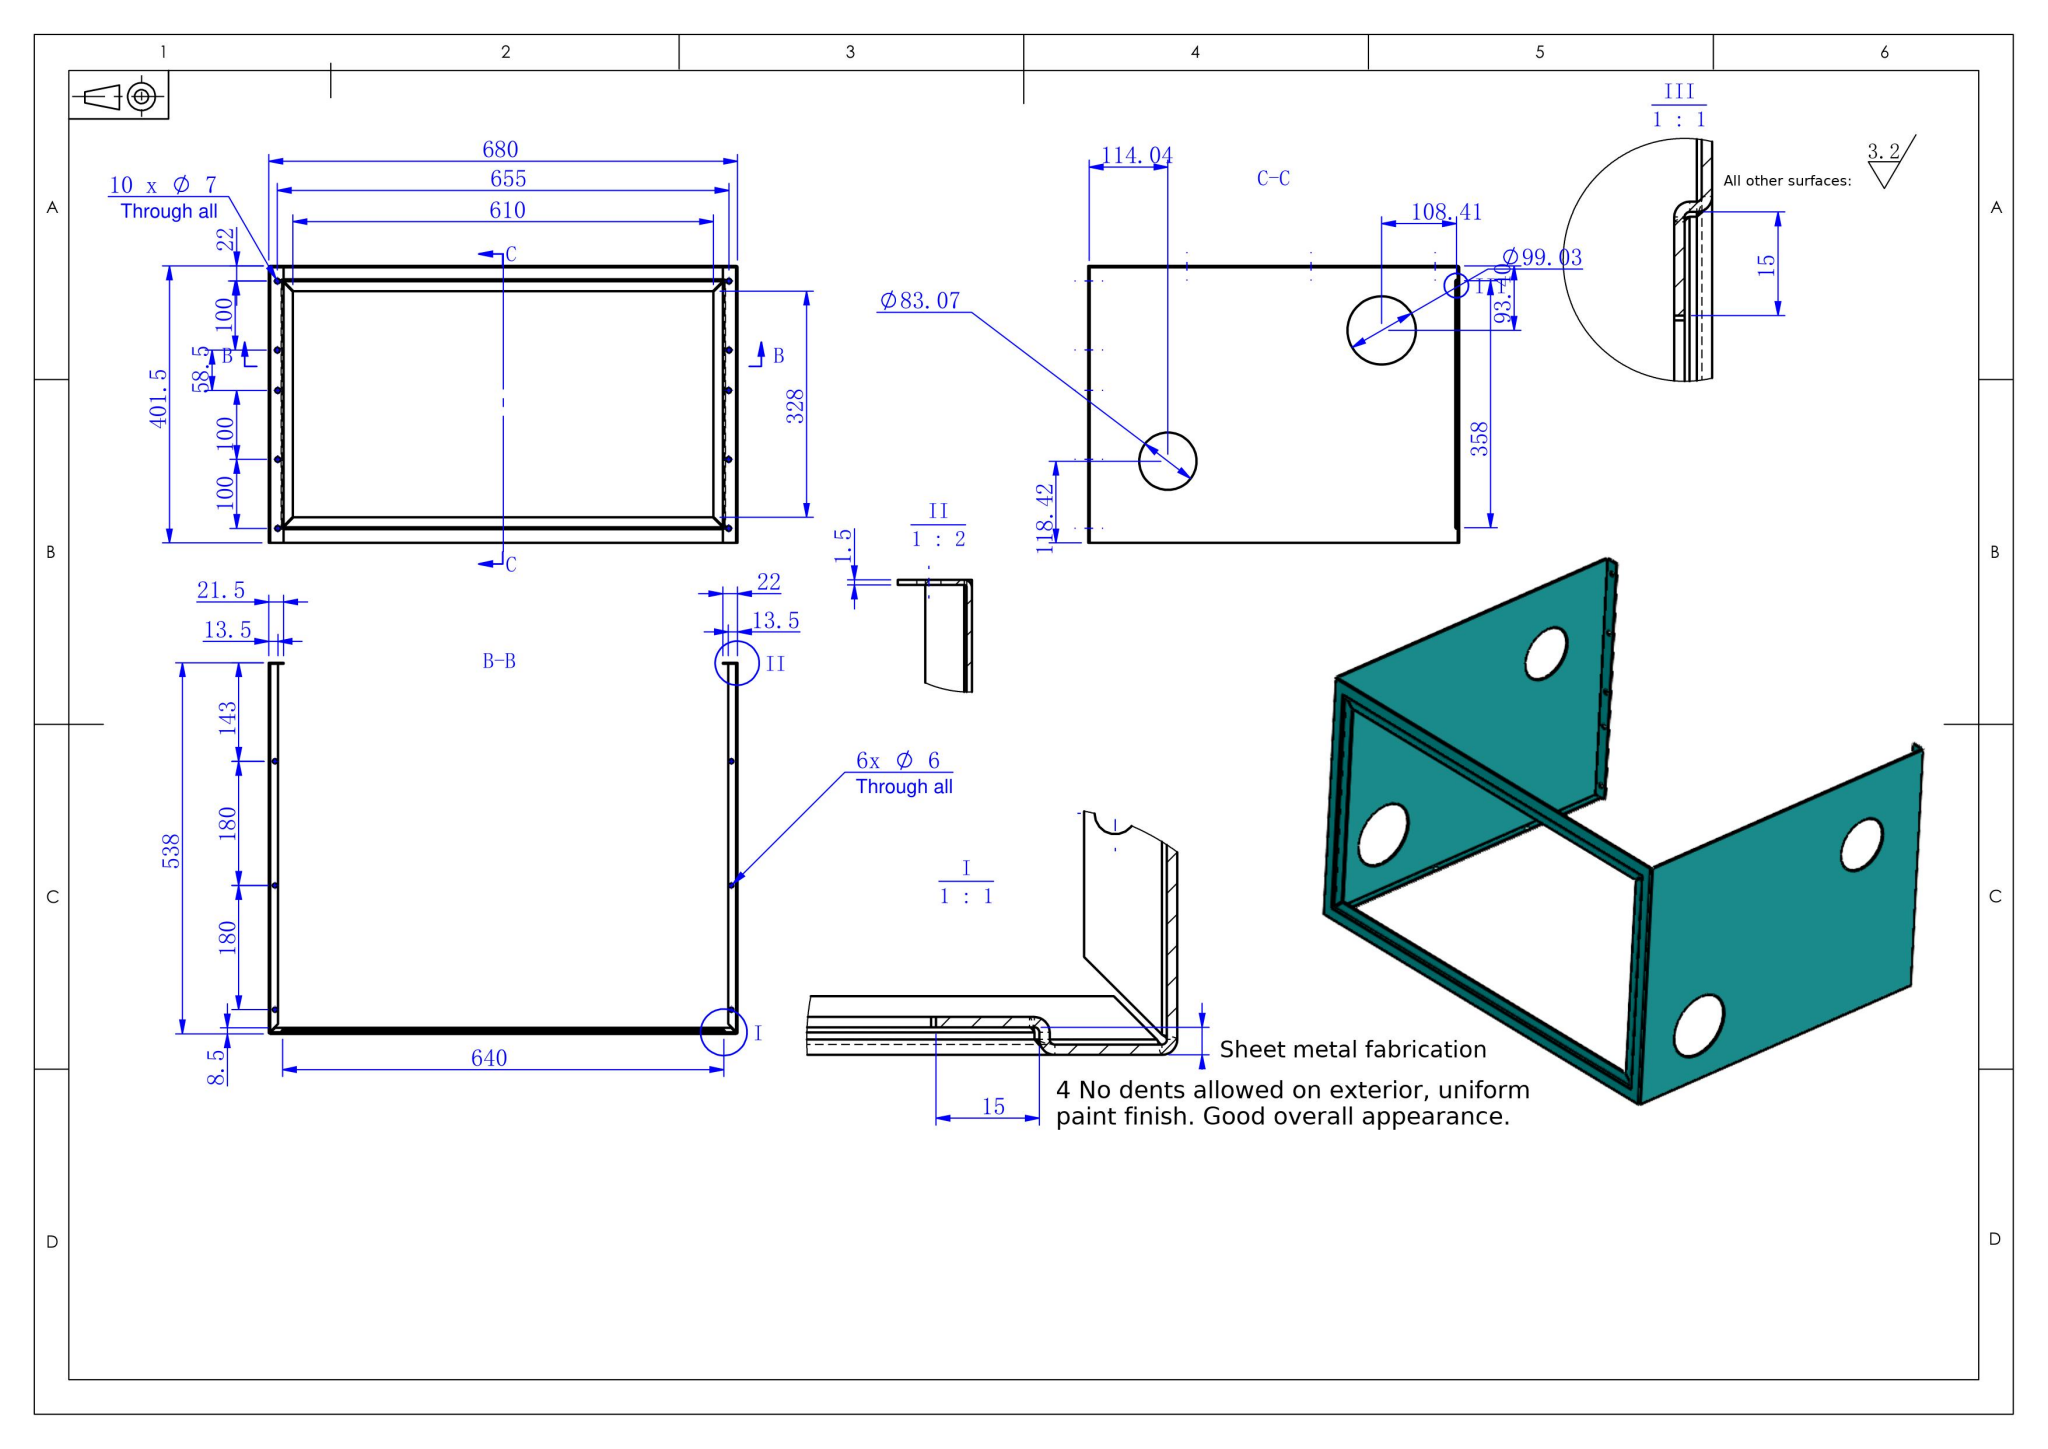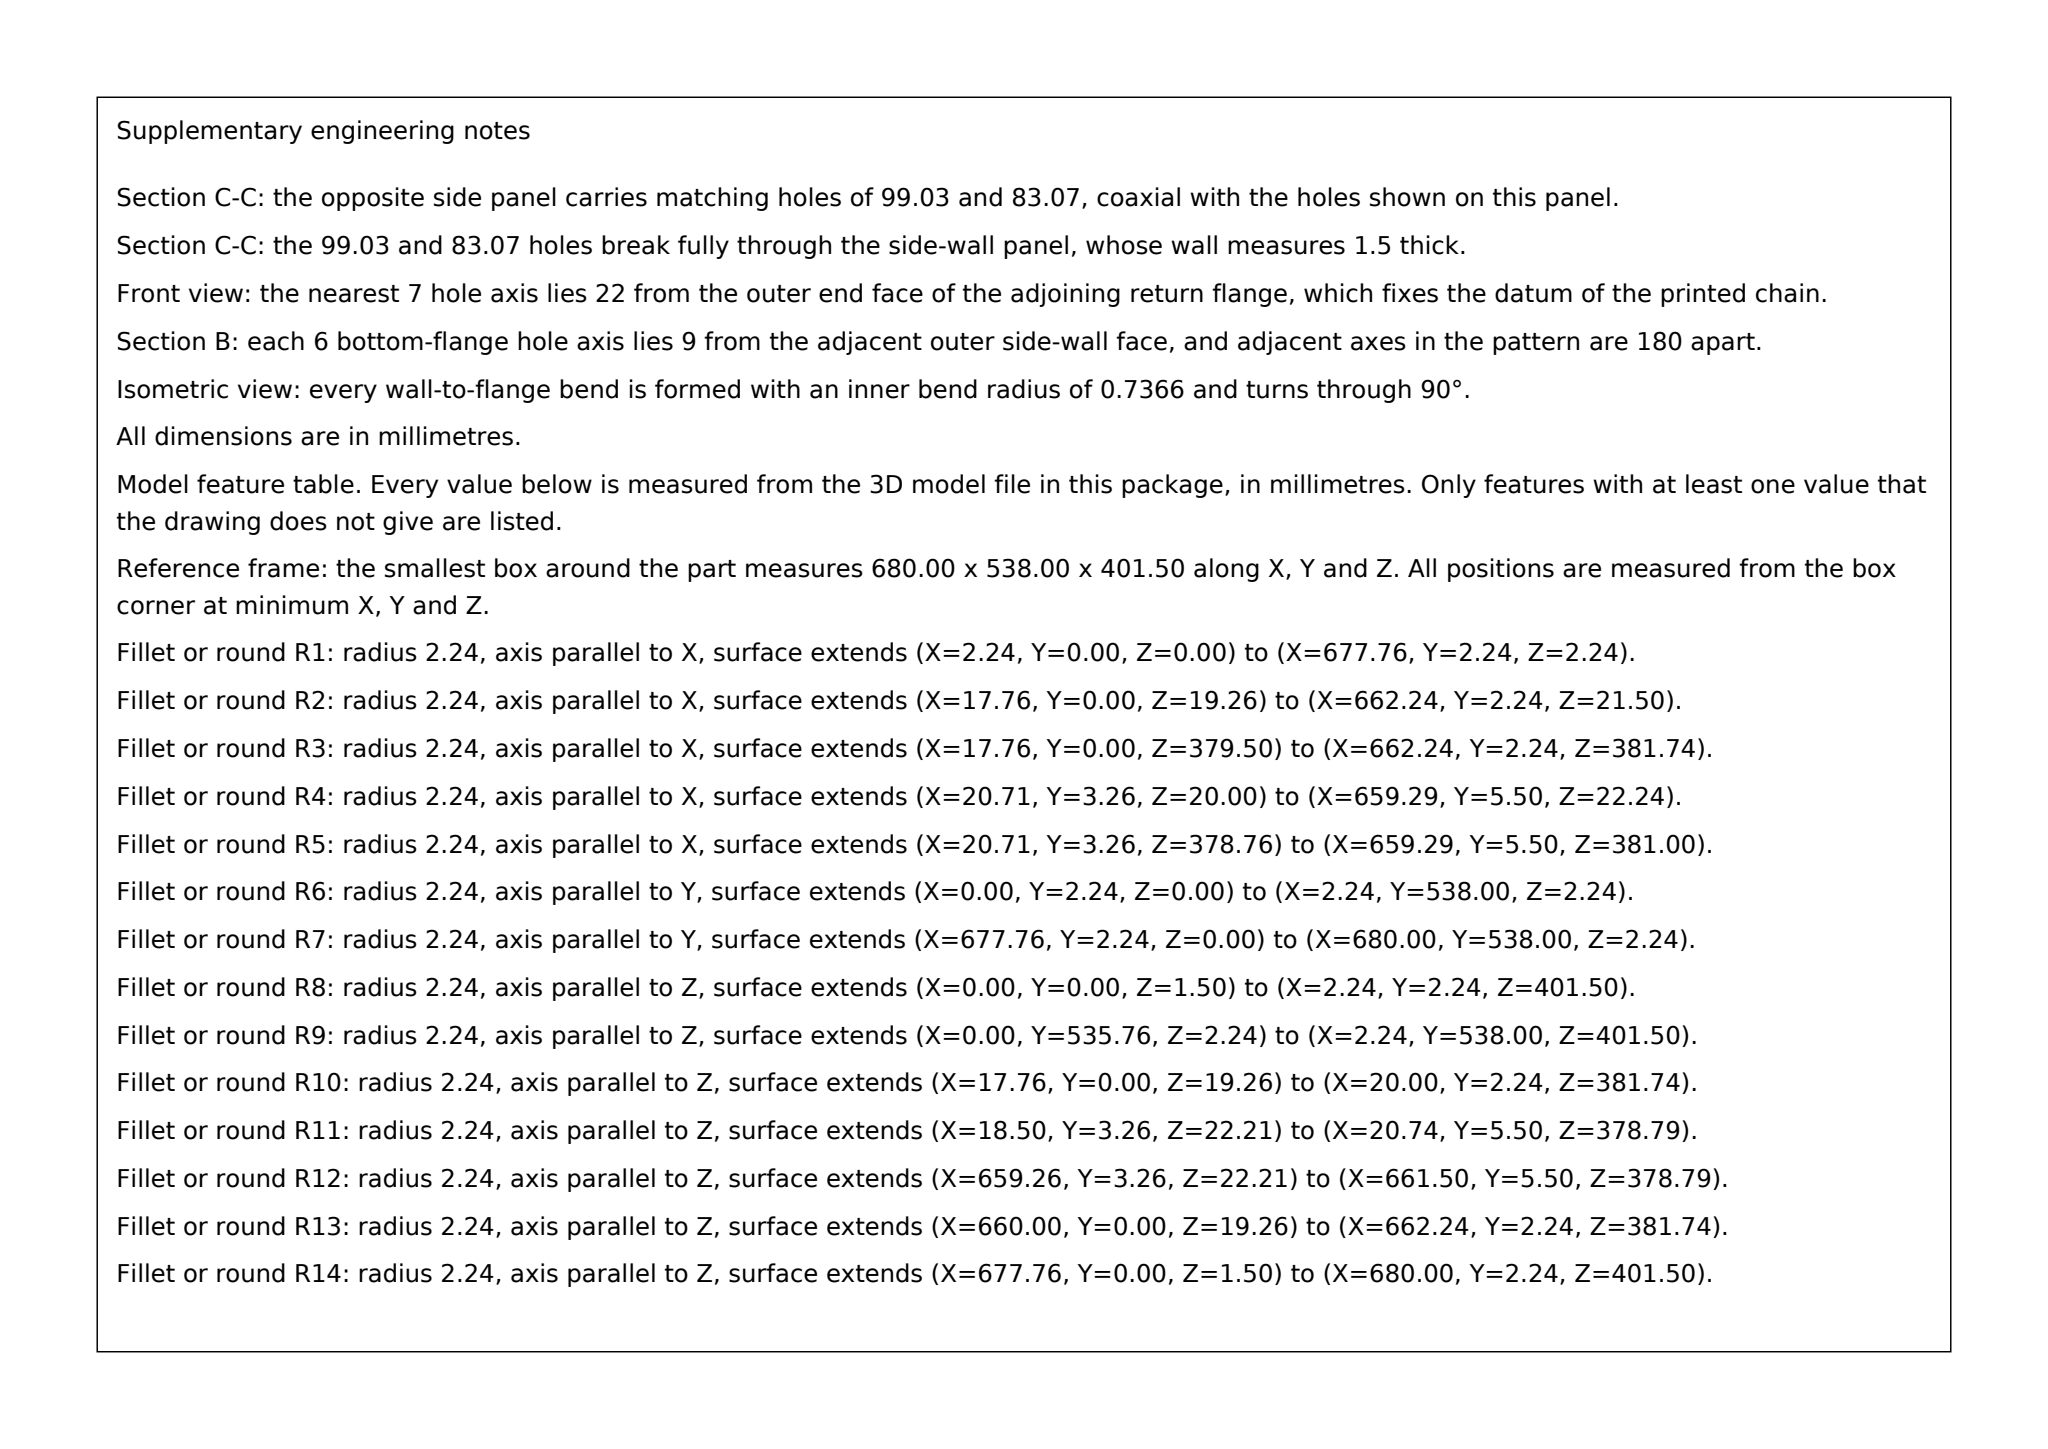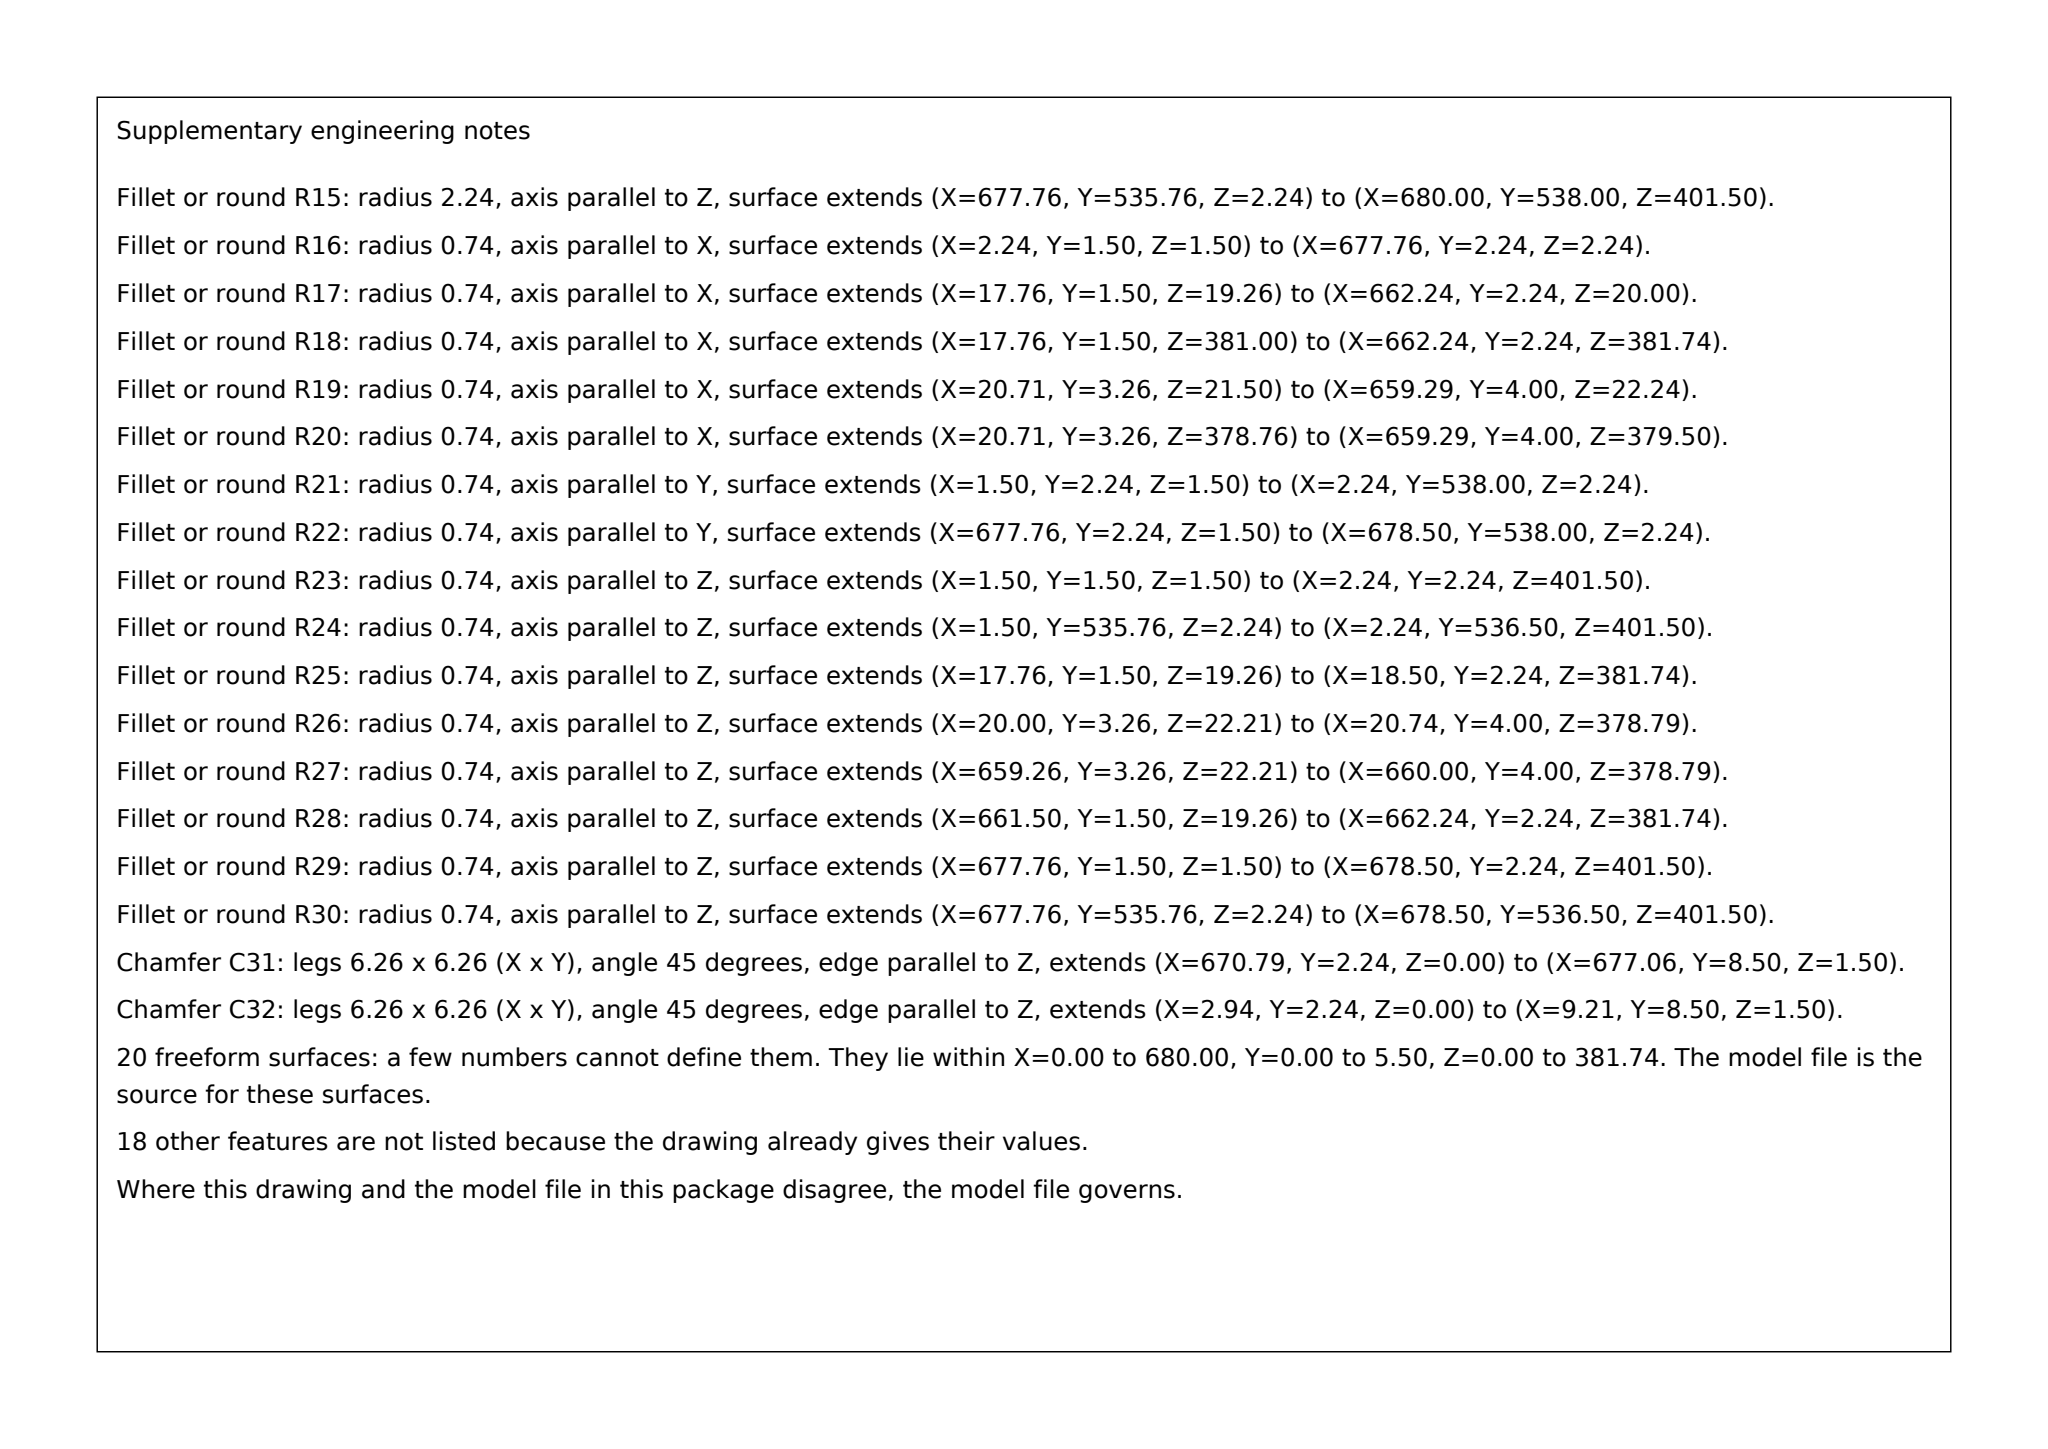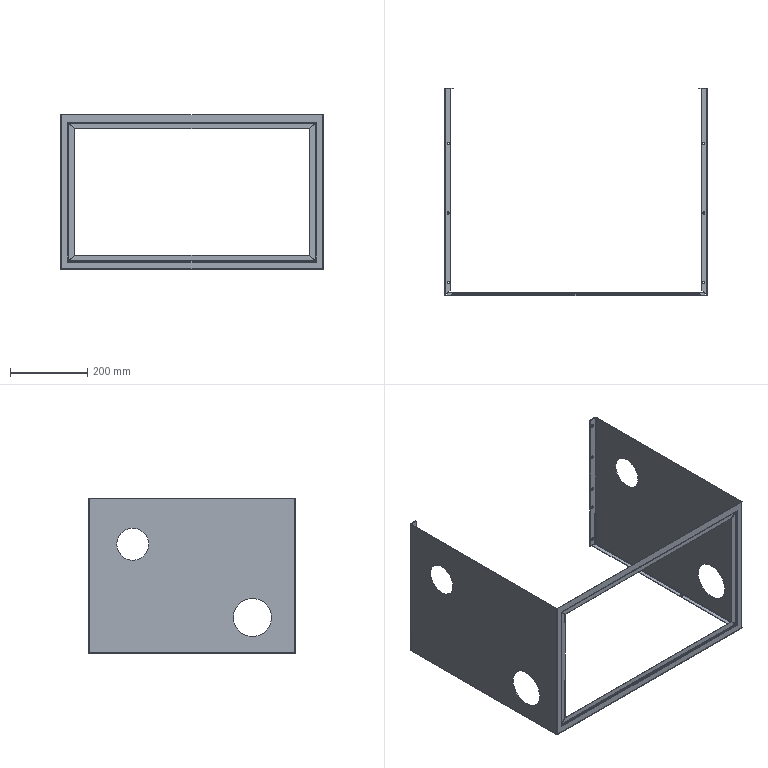Part | SolidWorks | mm | 1 solid | 176 faces | box 680 x 538 x 401.5 mm | volume 770247 mm3 | plane 86 | cylinder 70 | spline 20 | commonest cylinder face diameters 7 x20 4.473 x15 1.473 x15 6 x12 83.07 x4 99.026 x4
Drawing notes:
ALL BENDS (DET I/II/III): R0.74 INSIDE, R2.24 OUTSIDE, SHEET THK 1.5 | from the solid: Bend cylinders Ø1.473 (R0.737 inner) and Ø4.473 (R2.237 outer) on all flange edges; sheet thk 1.5 from plane offsets 0.02/1.52
2X Ø83.07 THRU (one in each side plate, mirrored about part centerline); hole axis parallel to X; center located 422.48 from the rear (min Y) face and 283.1 from the bottom (min Z) face. | from the solid: cylinders: [83.07,"x",[null,422.48,283.1],1.5,4] - through both side plates
2X Ø99.03 THRU (one in each side plate, mirrored about part centerline); hole axis parallel to X; center located 112.42 from the rear (min Y) face and 93.42 from the bottom (min Z) face. | from the solid: cylinders: [99.026,"x",[null,112.42,93.42],1.5,4] - through both side plates
6X Ø6 THRU in bottom plate: hole centers 9.02 from each side edge (X = 9.02 and X = 671.02) and at Y = 35.02, 215.02, 395.02 from the rear (min Y) face. | from the solid: cylinders: [6.0,"z",[9.02,35.02/215.02/395.02,null],1.5] and [6.0,"z",[671.02,35.02/215.02/395.02,null],1.5]
2X Ø83.07 THRU (1 in each side plate, mirrored about the part X centerline): hole center Y = 422.48, Z = 283.10 from the min-corner datum (bottom/front/left faces). | from the solid: cylinders entry [83.07,"x",[null,422.48,283.10],1.5] occurring 4 faces = 2 through holes, one per side plate
2X Ø99.03 THRU (1 in each side plate, mirrored about the part X centerline): hole center Y = 112.42, Z = 93.42 from the min-corner datum (bottom/front/left faces). | from the solid: cylinders entry [99.026,"x",[null,112.42,93.42],1.5] occurring 4 faces = 2 through holes, one per side plate
6X Ø6 THRU in the bottom plate: hole centers X = 9.02 from each long side edge (X = 9.02 and X = 671.02), Y = 35.02, 215.02 and 395.02 from the front edge. | from the solid: cylinders [6.0,"z",[9.02 / 671.02, 35.02 / 215.02 / 395.02],1.5] with bbox_xyz X = 680.03
6X Ø6 THRU in bottom plate (min Z face): hole centers at X = 9.02 and X = 671.02, Y = 35.02, 215.02 and 395.02 from min-corner datum (bottom/front/left faces). | from the solid: cylinders dia 6.0, axis z, positions [9.02/671.02, 35.02/215.02/395.02], length 1.5 (6 pairs)
10X Ø7 THRU in rear flange: hole centres at X = 12.52 and 667.52 (Z = 22.0 and 122.0) and X = 13.02 and 667.02 (Z = 180.5, 280.5, 380.5), all from the min-corner datum (bottom/front/left faces). | from the solid: cylinders: 10x 'hole/bore' dia 7.0, axis y, axis_pos (x,z) = (12.5,22.0),(12.5,122.0),(13.0,180.5),(13.0,280.5),(13.0,380.5),(667.5,22.0),(667.5,122.0),(667.0,180.5),(667.0,280.5),(667.0,380.5)
All 10X Ø7 holes lie in the rear flange only (flange material y = 536.5 to 538.0, THRU 1.5 thk); no Ø7 holes in the front flange. | from the solid: cylinders: all dia 7.0 bores have axis y with from 536.5 to 538.0; y-planes at 536.5 and 538.0, x [2.3,21.5] and [658.5,677.8]
Front-face return lip (sheet 1.5 thk, material between y = 4.0 and y = 5.5) forms a 14.2 wide ring: outer edges at X = 20.8 / 659.3 and Z = 22.2 / 378.8; inner edges at X = 35.02 / 645.02 and Z = 36.52 / 364.52 from the min-corner datum. | from the solid: axis_planes y=4.0 and y=5.5 with extents x[21.5,658.6] z[22.3,36.5] and z[364.5,378.8], x[20.8,35.0] and x[645.0,659.3] z[23.0,378.1]; x-planes at 35.0 and 645.0, y[4.0,5.5], z[37.2,363.8]
Bottom plate (z = 0 to 1.5) is a U-shaped strip: side strips X = 2.3 to 13.5 and X = 666.5 to 677.8 running Y = 3.0 to 538.0, joined by a front strip Y = 2.3 to 8.5 running X = 3.0 to 677.1 (centre open). | from the solid: z-planes at 0.0 and 1.5: x[2.3,13.5] y[3.0,538.0]; x[666.5,677.8] y[3.0,538.0]; x[3.0,677.1] y[2.3,8.5]
6X Ø6 THRU in bottom plate (plate Z = 0 to 1.5): hole centres at X = 9.0 and X = 671.0, Y = 35.0, 215.0 and 395.0 from the min-corner datum (bottom/front/left faces). | from the solid: hole/bore dia 6.0, axis z, at (9.0,35.0), (9.0,215.0), (9.0,395.0), (671.0,35.0), (671.0,215.0), (671.0,395.0), from z = 0.0 to 1.5
Bottom-plate side strips are 11.2 wide: X = 2.3 to 13.5 and X = 666.5 to 677.8, running Y = 3.0 to 538.0; Ø6 holes lie on these strips. | from the solid: axis_planes z = 0.0 / 1.5 with extent x [2.3,13.5] and x [666.5,677.8], y [3.0,538.0]